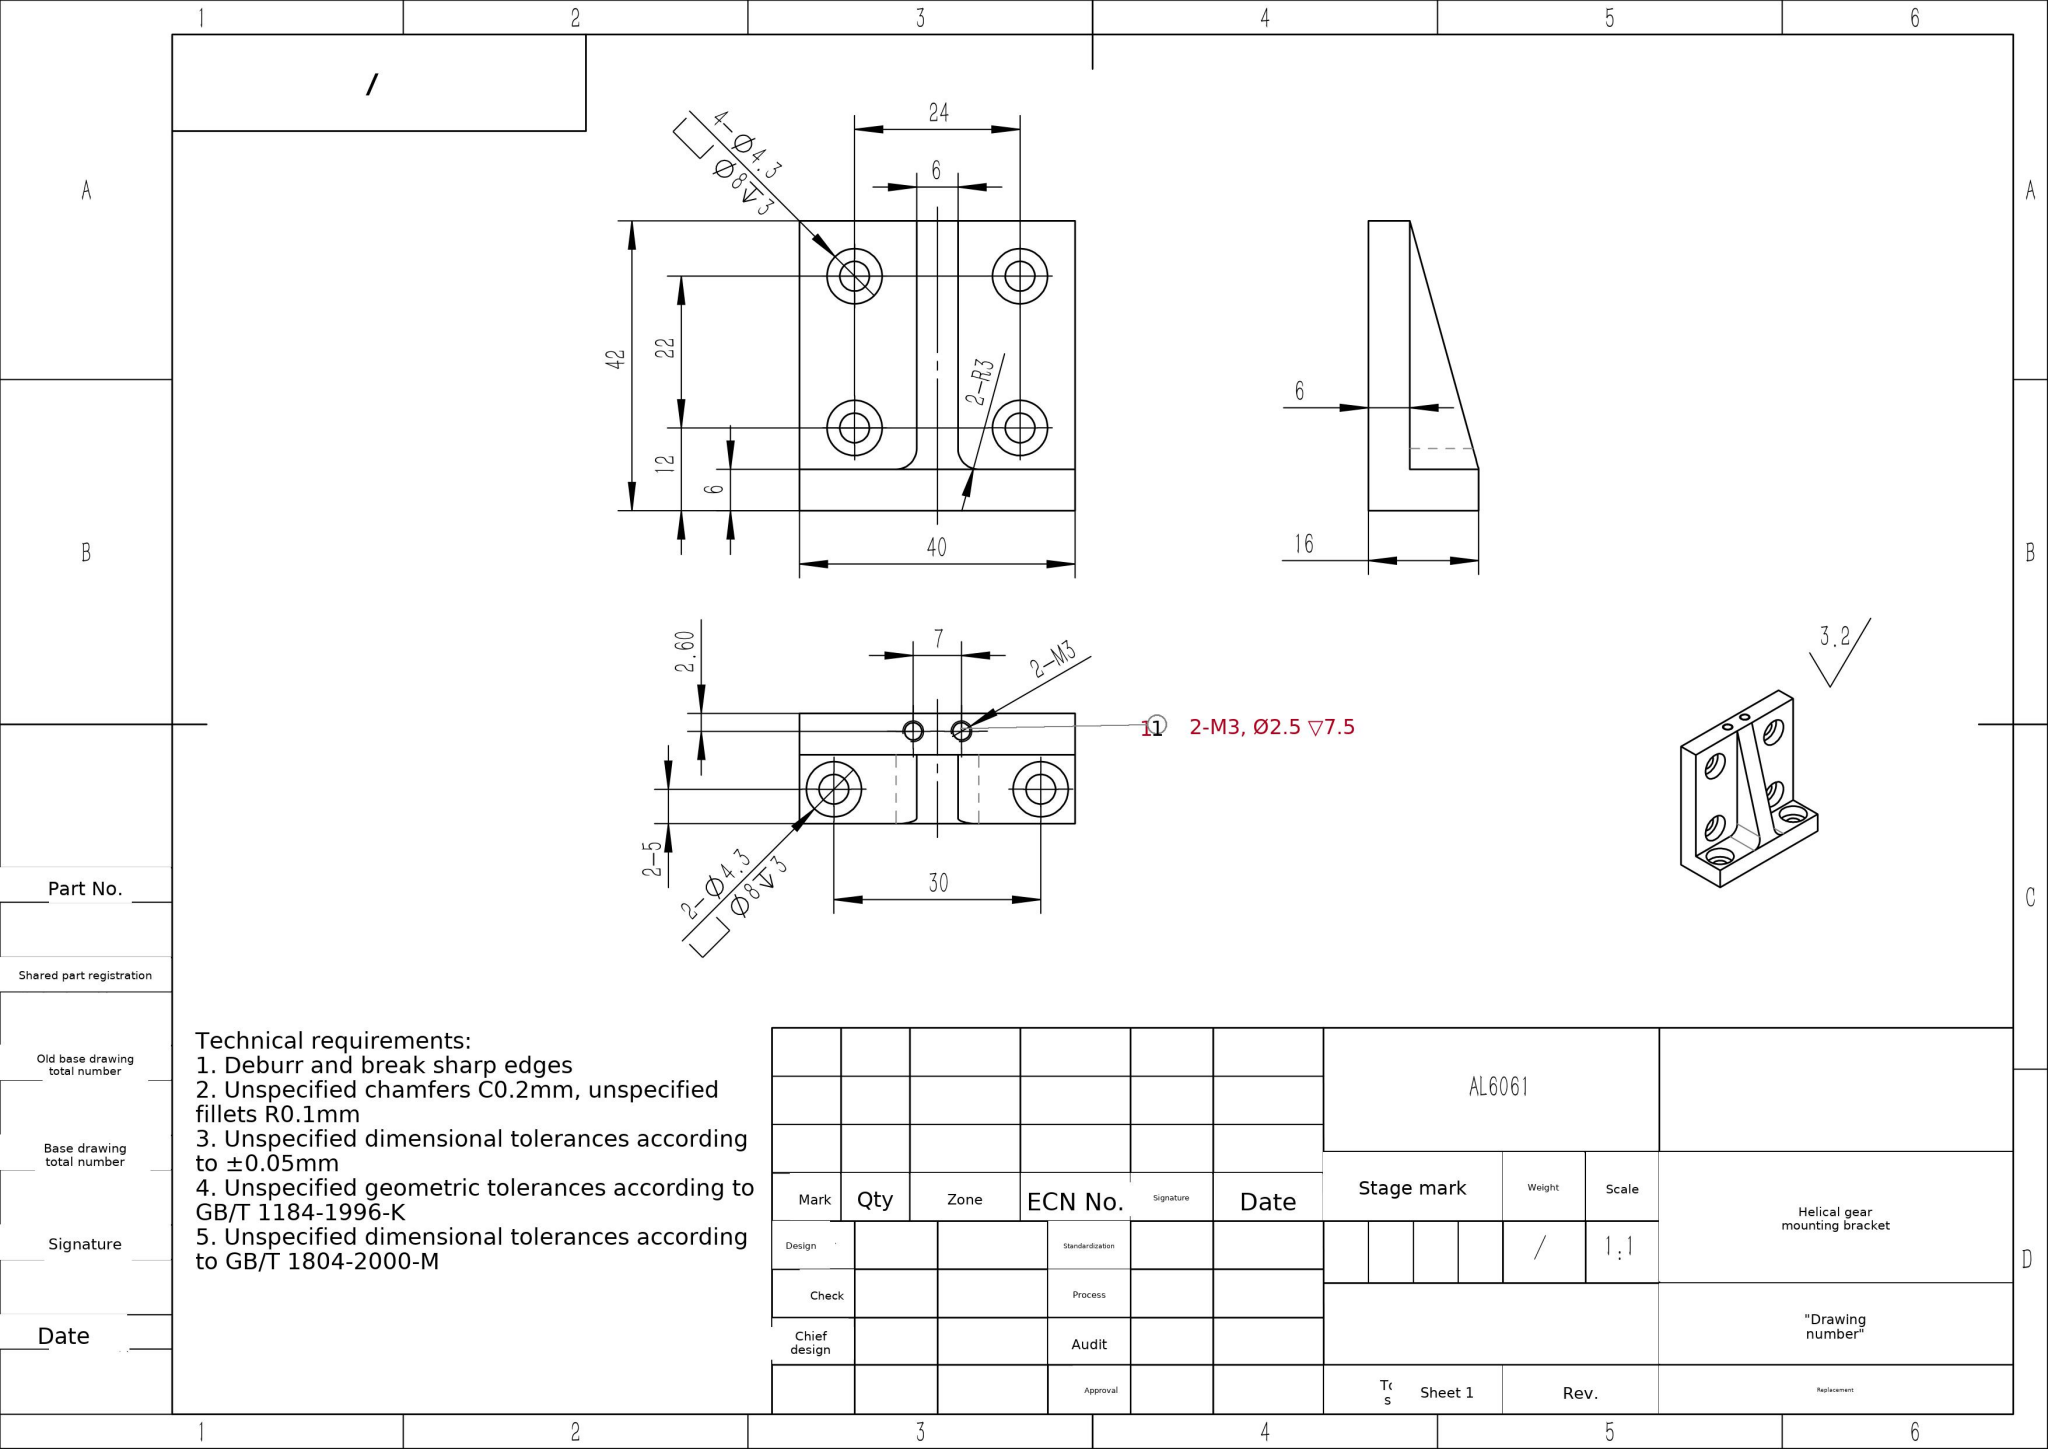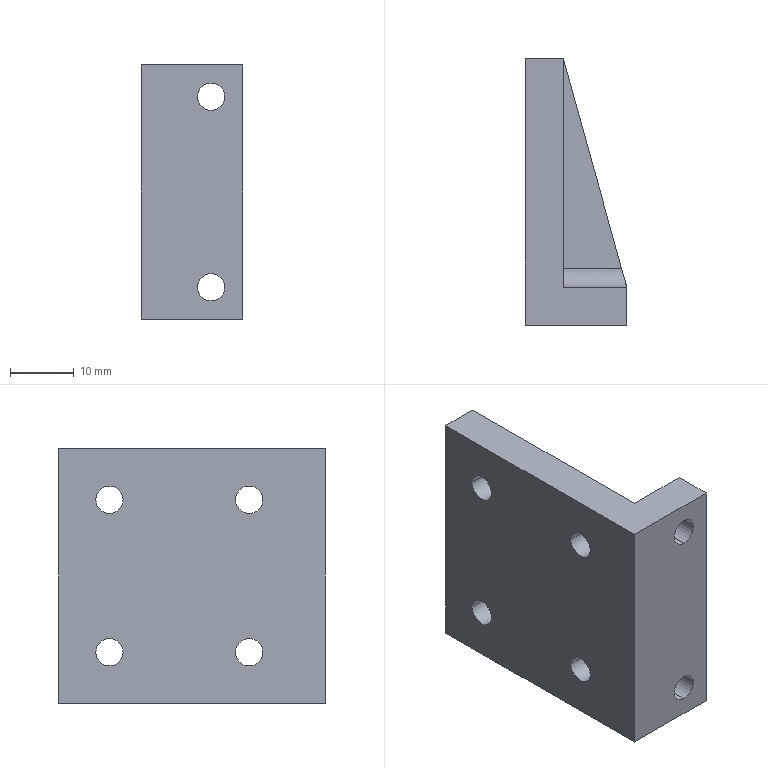Part | SolidWorks | mm | material AL6061 | 1 solid | 53 faces | box 16 x 42 x 40 mm | volume 12356 mm3 | cylinder 30 | plane 19 | cone 4 | commonest cylinder face diameters 8 x12 4.3 x12 2.5 x4 6 x2